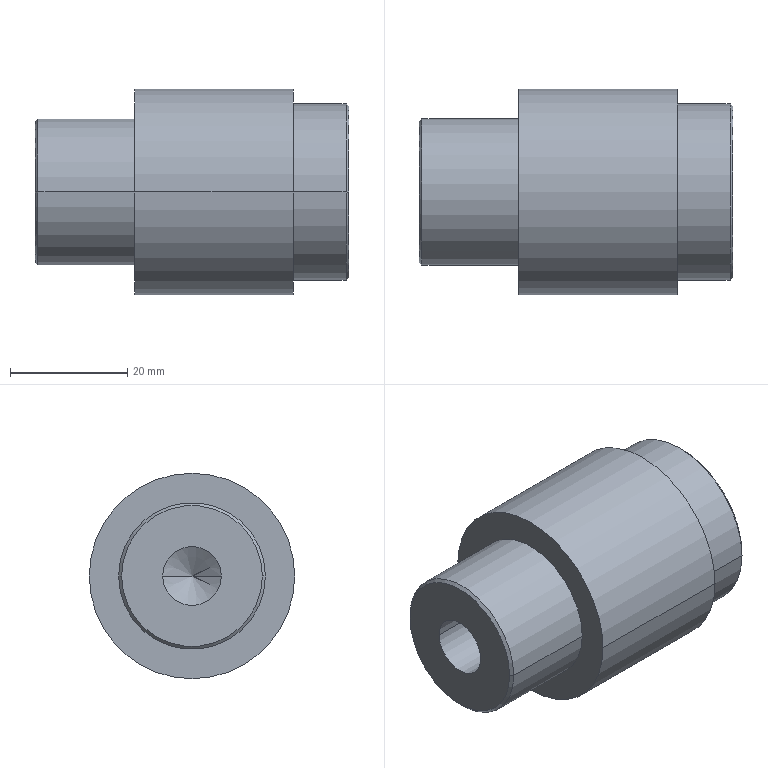Component | SolidWorks | GuideWheelAssembly-1_GuideWheelBracket-1_GuideWheelAxis-1 | 1 solid | 18 faces | box 53.5 x 35 x 35 mm | volume 39013 mm3 | cylinder 8 | cone 6 | plane 4 | commonest cylinder face diameters 10 x2 25 x2 35 x2 30 x2 | material Nylon 101
build123d program:
from build123d import *

# Parameters (mm, degrees)
SKETCH2_R              = 15
BOSS_EXTRUDE1_DEPTH    = 9.5
SKETCH3_R              = 17.5
BOSS_EXTRUDE2_DEPTH    = 27
SKETCH4_R              = 12.5
BOSS_EXTRUDE3_DEPTH    = 17
CHAMFER1_SIZE          = 0.5
M10_TAPPED_HOLE1_D     = 10
M10_TAPPED_HOLE1_DEPTH = 24.5
M10_TAPPED_HOLE1_TIP   = 3.004


with BuildPart() as part:
    # Sketch2 → Boss-Extrude1 (new body)
    with BuildSketch(Plane.XY):
        Circle(SKETCH2_R)
    extrude(amount=BOSS_EXTRUDE1_DEPTH)

    # Sketch3 → Boss-Extrude2 (add)
    with BuildSketch(Plane.XY.offset(9.5)):
        Circle(SKETCH3_R)
    extrude(amount=BOSS_EXTRUDE2_DEPTH)

    # Sketch4 → Boss-Extrude3 (add)
    with BuildSketch(Plane.XY.offset(36.5)):
        Circle(SKETCH4_R)
    extrude(amount=BOSS_EXTRUDE3_DEPTH)

    # Chamfer1
    chamfer1_edges = [part.edges().sort_by_distance(p)[0] for p in [
        (-12.5, 0, 53.5),
        (-15, 0, 0),
    ]]
    chamfer(chamfer1_edges, length=CHAMFER1_SIZE)

    # M10 Tapped Hole1
    with Locations(Plane.XY.offset(53.5)):
        with Locations((0, 0)):
            Hole(M10_TAPPED_HOLE1_D / 2, depth=M10_TAPPED_HOLE1_DEPTH)
            with Locations((0, 0, -(M10_TAPPED_HOLE1_DEPTH + M10_TAPPED_HOLE1_TIP / 2))):  # 118° drill point
                Cone(0, M10_TAPPED_HOLE1_D / 2, M10_TAPPED_HOLE1_TIP, mode=Mode.SUBTRACT)


solid = part.part

# Placed as in the assembly
solid = solid.moved(Location((-510.5, 0, 25), (0, -90, 0)))
STEP:
#1=COLOUR_RGB('',0.7922,0.8196,0.9333);
#2=FILL_AREA_STYLE_COLOUR('',#1);
#3=FILL_AREA_STYLE('',(#2));
#4=SURFACE_STYLE_FILL_AREA(#3);
#5=SURFACE_SIDE_STYLE('',(#4));
#6=SURFACE_STYLE_USAGE(.BOTH.,#5);
#7=PRESENTATION_STYLE_ASSIGNMENT((#6));
#8=CARTESIAN_POINT('',(-21.24,0.1969,0.9843));
#9=VERTEX_POINT('',#8);
#10=CARTESIAN_POINT('',(-21.24,-0.1969,0.9843));
#11=VERTEX_POINT('',#10);
#12=CARTESIAN_POINT('',(-21.24,-0.,0.9843));
#13=DIRECTION('',(-1.,0.,0.));
#14=DIRECTION('',(0.,-1.,0.));
#15=AXIS2_PLACEMENT_3D('',#12,#13,#14);
#16=CIRCLE('',#15,0.1969);
#17=EDGE_CURVE('',#9,#11,#16,.T.);
#18=ORIENTED_EDGE('',*,*,#17,.F.);
#19=CARTESIAN_POINT('',(-22.205,0.1969,0.9843));
#20=VERTEX_POINT('',#19);
#21=CARTESIAN_POINT('',(-22.205,0.1969,0.9843));
#22=DIRECTION('',(-1.,0.,0.));
#23=VECTOR('',#22,39.37);
#24=LINE('',#21,#23);
#25=EDGE_CURVE('',#9,#20,#24,.T.);
#26=ORIENTED_EDGE('',*,*,#25,.T.);
#27=CARTESIAN_POINT('',(-22.205,-0.1969,0.9843));
#28=VERTEX_POINT('',#27);
#29=CARTESIAN_POINT('',(-22.205,-0.,0.9843));
#30=DIRECTION('',(-1.,0.,0.));
#31=DIRECTION('',(0.,-1.,0.));
#32=AXIS2_PLACEMENT_3D('',#29,#30,#31);
#33=CIRCLE('',#32,0.1969);
#34=EDGE_CURVE('',#20,#28,#33,.T.);
#35=ORIENTED_EDGE('',*,*,#34,.T.);
#36=CARTESIAN_POINT('',(-22.205,-0.1969,0.9843));
#37=DIRECTION('',(-1.,0.,0.));
#38=VECTOR('',#37,39.37);
#39=LINE('',#36,#38);
#40=EDGE_CURVE('',#11,#28,#39,.T.);
#41=ORIENTED_EDGE('',*,*,#40,.F.);
#42=EDGE_LOOP('',(#18,#26,#35,#41));
#43=FACE_OUTER_BOUND('',#42,.T.);
#44=CARTESIAN_POINT('',(-22.205,-0.,0.9843));
#45=DIRECTION('',(-1.,0.,0.));
#46=DIRECTION('',(0.,-1.,0.));
#47=AXIS2_PLACEMENT_3D('',#44,#45,#46);
#48=CYLINDRICAL_SURFACE('',#47,0.1969);
#49=ADVANCED_FACE('',(#43),#48,.F.);
#50=CARTESIAN_POINT('',(-21.122,-0.,0.9843));
#51=VERTEX_POINT('',#50);
#52=CARTESIAN_POINT('',(-21.24,-0.1969,0.9843));
#53=DIRECTION('',(-0.515,-0.8572,0.));
#54=VECTOR('',#53,39.37);
#55=LINE('',#52,#54);
#56=EDGE_CURVE('',#51,#11,#55,.T.);
#57=ORIENTED_EDGE('',*,*,#56,.F.);
#58=CARTESIAN_POINT('',(-21.24,0.1969,0.9843));
#59=DIRECTION('',(-0.515,0.8572,0.));
#60=VECTOR('',#59,39.37);
#61=LINE('',#58,#60);
#62=EDGE_CURVE('',#51,#9,#61,.T.);
#63=ORIENTED_EDGE('',*,*,#62,.T.);
#64=ORIENTED_EDGE('',*,*,#17,.T.);
#65=EDGE_LOOP('',(#57,#63,#64));
#66=FACE_OUTER_BOUND('',#65,.T.);
#67=CARTESIAN_POINT('',(-21.24,-0.,0.9843));
#68=DIRECTION('',(-1.,0.,0.));
#69=DIRECTION('',(0.,-1.,0.));
#70=AXIS2_PLACEMENT_3D('',#67,#68,#69);
#71=CONICAL_SURFACE('',#70,0.1969,1.03);
#72=ADVANCED_FACE('',(#66),#71,.F.);
#73=CARTESIAN_POINT('',(-22.205,-0.4724,0.9843));
#74=VERTEX_POINT('',#73);
#75=CARTESIAN_POINT('',(-22.205,0.4724,0.9843));
#76=VERTEX_POINT('',#75);
#77=CARTESIAN_POINT('',(-22.205,-0.,0.9843));
#78=DIRECTION('',(-1.,0.,0.));
#79=DIRECTION('',(0.,-1.,0.));
#80=AXIS2_PLACEMENT_3D('',#77,#78,#79);
#81=CIRCLE('',#80,0.4724);
#82=EDGE_CURVE('',#74,#76,#81,.T.);
#83=ORIENTED_EDGE('',*,*,#82,.F.);
#84=CARTESIAN_POINT('',(-22.185,-0.4921,0.9843));
#85=VERTEX_POINT('',#84);
#86=CARTESIAN_POINT('',(-22.205,-0.4724,0.9843));
#87=DIRECTION('',(0.7071,-0.7071,0.));
#88=VECTOR('',#87,39.37);
#89=LINE('',#86,#88);
#90=EDGE_CURVE('',#74,#85,#89,.T.);
#91=ORIENTED_EDGE('',*,*,#90,.T.);
#92=CARTESIAN_POINT('',(-22.185,0.4921,0.9843));
#93=VERTEX_POINT('',#92);
#94=CARTESIAN_POINT('',(-22.185,-0.,0.9843));
#95=DIRECTION('',(1.,0.,0.));
#96=DIRECTION('',(0.,-1.,0.));
#97=AXIS2_PLACEMENT_3D('',#94,#95,#96);
#98=CIRCLE('',#97,0.4921);
#99=EDGE_CURVE('',#93,#85,#98,.T.);
#100=ORIENTED_EDGE('',*,*,#99,.F.);
#101=CARTESIAN_POINT('',(-22.205,0.4724,0.9843));
#102=DIRECTION('',(0.7071,0.7071,-0.));
#103=VECTOR('',#102,39.37);
#104=LINE('',#101,#103);
#105=EDGE_CURVE('',#76,#93,#104,.T.);
#106=ORIENTED_EDGE('',*,*,#105,.F.);
#107=EDGE_LOOP('',(#83,#91,#100,#106));
#108=FACE_OUTER_BOUND('',#107,.T.);
#109=CARTESIAN_POINT('',(-22.205,-0.,0.9843));
#110=DIRECTION('',(1.,0.,0.));
#111=DIRECTION('',(0.,1.,0.));
#112=AXIS2_PLACEMENT_3D('',#109,#110,#111);
#113=CONICAL_SURFACE('',#112,0.4724,0.7854);
#114=ADVANCED_FACE('',(#108),#113,.T.);
#115=CARTESIAN_POINT('',(-20.098,0.5709,0.9843));
#116=VERTEX_POINT('',#115);
#117=CARTESIAN_POINT('',(-20.098,-0.5709,0.9843));
#118=VERTEX_POINT('',#117);
#119=CARTESIAN_POINT('',(-20.098,-0.,0.9843));
#120=DIRECTION('',(1.,0.,0.));
#121=DIRECTION('',(0.,-1.,0.));
#122=AXIS2_PLACEMENT_3D('',#119,#120,#121);
#123=CIRCLE('',#122,0.5709);
#124=EDGE_CURVE('',#116,#118,#123,.T.);
#125=ORIENTED_EDGE('',*,*,#124,.F.);
#126=CARTESIAN_POINT('',(-20.118,0.5906,0.9843));
#127=VERTEX_POINT('',#126);
#128=CARTESIAN_POINT('',(-20.118,0.5906,0.9843));
#129=DIRECTION('',(-0.7071,0.7071,0.));
#130=VECTOR('',#129,39.37);
#131=LINE('',#128,#130);
#132=EDGE_CURVE('',#116,#127,#131,.T.);
#133=ORIENTED_EDGE('',*,*,#132,.T.);
#134=CARTESIAN_POINT('',(-20.118,-0.5906,0.9843));
#135=VERTEX_POINT('',#134);
#136=CARTESIAN_POINT('',(-20.118,-0.,0.9843));
#137=DIRECTION('',(-1.,0.,0.));
#138=DIRECTION('',(0.,-1.,0.));
#139=AXIS2_PLACEMENT_3D('',#136,#137,#138);
#140=CIRCLE('',#139,0.5906);
#141=EDGE_CURVE('',#135,#127,#140,.T.);
#142=ORIENTED_EDGE('',*,*,#141,.F.);
#143=CARTESIAN_POINT('',(-20.118,-0.5906,0.9843));
#144=DIRECTION('',(-0.7071,-0.7071,0.));
#145=VECTOR('',#144,39.37);
#146=LINE('',#143,#145);
#147=EDGE_CURVE('',#118,#135,#146,.T.);
#148=ORIENTED_EDGE('',*,*,#147,.F.);
#149=EDGE_LOOP('',(#125,#133,#142,#148));
#150=FACE_OUTER_BOUND('',#149,.T.);
#151=CARTESIAN_POINT('',(-20.118,-0.,0.9843));
#152=DIRECTION('',(-1.,0.,0.));
#153=DIRECTION('',(0.,-1.,0.));
#154=AXIS2_PLACEMENT_3D('',#151,#152,#153);
#155=CONICAL_SURFACE('',#154,0.5906,0.7854);
#156=ADVANCED_FACE('',(#150),#155,.T.);
#157=ORIENTED_EDGE('',*,*,#99,.T.);
#158=CARTESIAN_POINT('',(-21.535,-0.4921,0.9843));
#159=VERTEX_POINT('',#158);
#160=CARTESIAN_POINT('',(-22.205,-0.4921,0.9843));
#161=DIRECTION('',(1.,0.,0.));
#162=VECTOR('',#161,39.37);
#163=LINE('',#160,#162);
#164=EDGE_CURVE('',#85,#159,#163,.T.);
#165=ORIENTED_EDGE('',*,*,#164,.T.);
#166=CARTESIAN_POINT('',(-21.535,0.4921,0.9843));
#167=VERTEX_POINT('',#166);
#168=CARTESIAN_POINT('',(-21.535,-0.,0.9843));
#169=DIRECTION('',(-1.,0.,0.));
#170=DIRECTION('',(0.,-1.,0.));
#171=AXIS2_PLACEMENT_3D('',#168,#169,#170);
#172=CIRCLE('',#171,0.4921);
#173=EDGE_CURVE('',#159,#167,#172,.T.);
#174=ORIENTED_EDGE('',*,*,#173,.T.);
#175=CARTESIAN_POINT('',(-22.205,0.4921,0.9843));
#176=DIRECTION('',(1.,0.,0.));
#177=VECTOR('',#176,39.37);
#178=LINE('',#175,#177);
#179=EDGE_CURVE('',#93,#167,#178,.T.);
#180=ORIENTED_EDGE('',*,*,#179,.F.);
#181=EDGE_LOOP('',(#157,#165,#174,#180));
#182=FACE_OUTER_BOUND('',#181,.T.);
#183=CARTESIAN_POINT('',(-22.205,-0.,0.9843));
#184=DIRECTION('',(1.,0.,0.));
#185=DIRECTION('',(0.,1.,0.));
#186=AXIS2_PLACEMENT_3D('',#183,#184,#185);
#187=CYLINDRICAL_SURFACE('',#186,0.4921);
#188=ADVANCED_FACE('',(#182),#187,.T.);
#189=CARTESIAN_POINT('',(-21.535,-0.689,0.9843));
#190=VERTEX_POINT('',#189);
#191=CARTESIAN_POINT('',(-21.535,0.689,0.9843));
#192=VERTEX_POINT('',#191);
#193=CARTESIAN_POINT('',(-21.535,-0.,0.9843));
#194=DIRECTION('',(-1.,0.,0.));
#195=DIRECTION('',(0.,-1.,0.));
#196=AXIS2_PLACEMENT_3D('',#193,#194,#195);
#197=CIRCLE('',#196,0.689);
#198=EDGE_CURVE('',#190,#192,#197,.T.);
#199=ORIENTED_EDGE('',*,*,#198,.F.);
#200=CARTESIAN_POINT('',(-20.472,-0.689,0.9843));
#201=VERTEX_POINT('',#200);
#202=CARTESIAN_POINT('',(-21.535,-0.689,0.9843));
#203=DIRECTION('',(1.,0.,0.));
#204=VECTOR('',#203,39.37);
#205=LINE('',#202,#204);
#206=EDGE_CURVE('',#190,#201,#205,.T.);
#207=ORIENTED_EDGE('',*,*,#206,.T.);
#208=CARTESIAN_POINT('',(-20.472,0.689,0.9843));
#209=VERTEX_POINT('',#208);
#210=CARTESIAN_POINT('',(-20.472,-0.,0.9843));
#211=DIRECTION('',(-1.,0.,0.));
#212=DIRECTION('',(0.,-1.,0.));
#213=AXIS2_PLACEMENT_3D('',#210,#211,#212);
#214=CIRCLE('',#213,0.689);
#215=EDGE_CURVE('',#201,#209,#214,.T.);
#216=ORIENTED_EDGE('',*,*,#215,.T.);
#217=CARTESIAN_POINT('',(-21.535,0.689,0.9843));
#218=DIRECTION('',(1.,0.,0.));
#219=VECTOR('',#218,39.37);
#220=LINE('',#217,#219);
#221=EDGE_CURVE('',#192,#209,#220,.T.);
#222=ORIENTED_EDGE('',*,*,#221,.F.);
#223=EDGE_LOOP('',(#199,#207,#216,#222));
#224=FACE_OUTER_BOUND('',#223,.T.);
#225=CARTESIAN_POINT('',(-21.535,-0.,0.9843));
#226=DIRECTION('',(1.,0.,0.));
#227=DIRECTION('',(0.,1.,-0.));
#228=AXIS2_PLACEMENT_3D('',#225,#226,#227);
#229=CYLINDRICAL_SURFACE('',#228,0.689);
#230=ADVANCED_FACE('',(#224),#229,.T.);
#231=CARTESIAN_POINT('',(-20.472,-0.5906,0.9843));
#232=VERTEX_POINT('',#231);
#233=CARTESIAN_POINT('',(-20.472,0.5906,0.9843));
#234=VERTEX_POINT('',#233);
#235=CARTESIAN_POINT('',(-20.472,-0.,0.9843));
#236=DIRECTION('',(-1.,0.,0.));
#237=DIRECTION('',(0.,-1.,0.));
#238=AXIS2_PLACEMENT_3D('',#235,#236,#237);
#239=CIRCLE('',#238,0.5906);
#240=EDGE_CURVE('',#232,#234,#239,.T.);
#241=ORIENTED_EDGE('',*,*,#240,.F.);
#242=CARTESIAN_POINT('',(-20.472,-0.5906,0.9843));
#243=DIRECTION('',(1.,0.,0.));
#244=VECTOR('',#243,39.37);
#245=LINE('',#242,#244);
#246=EDGE_CURVE('',#232,#135,#245,.T.);
#247=ORIENTED_EDGE('',*,*,#246,.T.);
#248=ORIENTED_EDGE('',*,*,#141,.T.);
#249=CARTESIAN_POINT('',(-20.472,0.5906,0.9843));
#250=DIRECTION('',(1.,0.,0.));
#251=VECTOR('',#250,39.37);
#252=LINE('',#249,#251);
#253=EDGE_CURVE('',#234,#127,#252,.T.);
#254=ORIENTED_EDGE('',*,*,#253,.F.);
#255=EDGE_LOOP('',(#241,#247,#248,#254));
#256=FACE_OUTER_BOUND('',#255,.T.);
#257=CARTESIAN_POINT('',(-20.472,-0.,0.9843));
#258=DIRECTION('',(1.,0.,0.));
#259=DIRECTION('',(0.,1.,0.));
#260=AXIS2_PLACEMENT_3D('',#257,#258,#259);
#261=CYLINDRICAL_SURFACE('',#260,0.5906);
#262=ADVANCED_FACE('',(#256),#261,.T.);
#263=CARTESIAN_POINT('',(-21.535,-0.,0.9843));
#264=DIRECTION('',(-1.,0.,0.));
#265=DIRECTION('',(0.,-1.,0.));
#266=AXIS2_PLACEMENT_3D('',#263,#264,#265);
#267=CIRCLE('',#266,0.689);
#268=EDGE_CURVE('',#192,#190,#267,.T.);
#269=ORIENTED_EDGE('',*,*,#268,.T.);
#270=ORIENTED_EDGE('',*,*,#198,.T.);
#271=EDGE_LOOP('',(#269,#270));
#272=FACE_OUTER_BOUND('',#271,.T.);
#273=CARTESIAN_POINT('',(-21.535,-0.,0.9843));
#274=DIRECTION('',(-1.,0.,0.));
#275=DIRECTION('',(0.,-1.,0.));
#276=AXIS2_PLACEMENT_3D('',#273,#274,#275);
#277=CIRCLE('',#276,0.4921);
#278=EDGE_CURVE('',#167,#159,#277,.T.);
#279=ORIENTED_EDGE('',*,*,#278,.F.);
#280=ORIENTED_EDGE('',*,*,#173,.F.);
#281=EDGE_LOOP('',(#279,#280));
#282=FACE_BOUND('',#281,.T.);
#283=CARTESIAN_POINT('',(-21.535,-0.,0.9843));
#284=DIRECTION('',(-1.,0.,0.));
#285=DIRECTION('',(0.,-1.,0.));
#286=AXIS2_PLACEMENT_3D('',#283,#284,#285);
#287=PLANE('',#286);
#288=ADVANCED_FACE('',(#272,#282),#287,.T.);
#289=ORIENTED_EDGE('',*,*,#246,.F.);
#290=CARTESIAN_POINT('',(-20.472,-0.,0.9843));
#291=DIRECTION('',(-1.,0.,0.));
#292=DIRECTION('',(0.,-1.,0.));
#293=AXIS2_PLACEMENT_3D('',#290,#291,#292);
#294=CIRCLE('',#293,0.5906);
#295=EDGE_CURVE('',#234,#232,#294,.T.);
#296=ORIENTED_EDGE('',*,*,#295,.F.);
#297=ORIENTED_EDGE('',*,*,#253,.T.);
#298=CARTESIAN_POINT('',(-20.118,-0.,0.9843));
#299=DIRECTION('',(-1.,0.,0.));
#300=DIRECTION('',(0.,-1.,0.));
#301=AXIS2_PLACEMENT_3D('',#298,#299,#300);
#302=CIRCLE('',#301,0.5906);
#303=EDGE_CURVE('',#127,#135,#302,.T.);
#304=ORIENTED_EDGE('',*,*,#303,.T.);
#305=EDGE_LOOP('',(#289,#296,#297,#304));
#306=FACE_OUTER_BOUND('',#305,.T.);
#307=CARTESIAN_POINT('',(-20.472,-0.,0.9843));
#308=DIRECTION('',(1.,0.,0.));
#309=DIRECTION('',(0.,1.,0.));
#310=AXIS2_PLACEMENT_3D('',#307,#308,#309);
#311=CYLINDRICAL_SURFACE('',#310,0.5906);
#312=ADVANCED_FACE('',(#306),#311,.T.);
#313=CARTESIAN_POINT('',(-20.098,-0.,0.9843));
#314=DIRECTION('',(1.,0.,0.));
#315=DIRECTION('',(0.,-1.,0.));
#316=AXIS2_PLACEMENT_3D('',#313,#314,#315);
#317=CIRCLE('',#316,0.5709);
#318=EDGE_CURVE('',#118,#116,#317,.T.);
#319=ORIENTED_EDGE('',*,*,#318,.T.);
#320=ORIENTED_EDGE('',*,*,#124,.T.);
#321=EDGE_LOOP('',(#319,#320));
#322=FACE_OUTER_BOUND('',#321,.T.);
#323=CARTESIAN_POINT('',(-20.098,-0.,0.9843));
#324=DIRECTION('',(-1.,0.,0.));
#325=DIRECTION('',(0.,-1.,0.));
#326=AXIS2_PLACEMENT_3D('',#323,#324,#325);
#327=PLANE('',#326);
#328=ADVANCED_FACE('',(#322),#327,.F.);
#329=CARTESIAN_POINT('',(-20.472,-0.,0.9843));
#330=DIRECTION('',(-1.,0.,0.));
#331=DIRECTION('',(0.,-1.,0.));
#332=AXIS2_PLACEMENT_3D('',#329,#330,#331);
#333=CIRCLE('',#332,0.689);
#334=EDGE_CURVE('',#209,#201,#333,.T.);
#335=ORIENTED_EDGE('',*,*,#334,.F.);
#336=ORIENTED_EDGE('',*,*,#215,.F.);
#337=EDGE_LOOP('',(#335,#336));
#338=FACE_OUTER_BOUND('',#337,.T.);
#339=ORIENTED_EDGE('',*,*,#295,.T.);
#340=ORIENTED_EDGE('',*,*,#240,.T.);
#341=EDGE_LOOP('',(#339,#340));
#342=FACE_BOUND('',#341,.T.);
#343=CARTESIAN_POINT('',(-20.472,-0.,0.9843));
#344=DIRECTION('',(-1.,0.,0.));
#345=DIRECTION('',(0.,-1.,0.));
#346=AXIS2_PLACEMENT_3D('',#343,#344,#345);
#347=PLANE('',#346);
#348=ADVANCED_FACE('',(#338,#342),#347,.F.);
#349=ORIENTED_EDGE('',*,*,#206,.F.);
#350=ORIENTED_EDGE('',*,*,#268,.F.);
#351=ORIENTED_EDGE('',*,*,#221,.T.);
#352=ORIENTED_EDGE('',*,*,#334,.T.);
#353=EDGE_LOOP('',(#349,#350,#351,#352));
#354=FACE_OUTER_BOUND('',#353,.T.);
#355=CARTESIAN_POINT('',(-21.535,-0.,0.9843));
#356=DIRECTION('',(1.,0.,0.));
#357=DIRECTION('',(0.,1.,-0.));
#358=AXIS2_PLACEMENT_3D('',#355,#356,#357);
#359=CYLINDRICAL_SURFACE('',#358,0.689);
#360=ADVANCED_FACE('',(#354),#359,.T.);
#361=ORIENTED_EDGE('',*,*,#164,.F.);
#362=CARTESIAN_POINT('',(-22.185,-0.,0.9843));
#363=DIRECTION('',(1.,0.,0.));
#364=DIRECTION('',(0.,-1.,0.));
#365=AXIS2_PLACEMENT_3D('',#362,#363,#364);
#366=CIRCLE('',#365,0.4921);
#367=EDGE_CURVE('',#85,#93,#366,.T.);
#368=ORIENTED_EDGE('',*,*,#367,.T.);
#369=ORIENTED_EDGE('',*,*,#179,.T.);
#370=ORIENTED_EDGE('',*,*,#278,.T.);
#371=EDGE_LOOP('',(#361,#368,#369,#370));
#372=FACE_OUTER_BOUND('',#371,.T.);
#373=CARTESIAN_POINT('',(-22.205,-0.,0.9843));
#374=DIRECTION('',(1.,0.,0.));
#375=DIRECTION('',(0.,1.,0.));
#376=AXIS2_PLACEMENT_3D('',#373,#374,#375);
#377=CYLINDRICAL_SURFACE('',#376,0.4921);
#378=ADVANCED_FACE('',(#372),#377,.T.);
#379=CARTESIAN_POINT('',(-22.205,-0.,0.9843));
#380=DIRECTION('',(-1.,0.,0.));
#381=DIRECTION('',(0.,-1.,0.));
#382=AXIS2_PLACEMENT_3D('',#379,#380,#381);
#383=CIRCLE('',#382,0.1969);
#384=EDGE_CURVE('',#28,#20,#383,.T.);
#385=ORIENTED_EDGE('',*,*,#384,.F.);
#386=ORIENTED_EDGE('',*,*,#34,.F.);
#387=EDGE_LOOP('',(#385,#386));
#388=FACE_BOUND('',#387,.T.);
#389=CARTESIAN_POINT('',(-22.205,-0.,0.9843));
#390=DIRECTION('',(-1.,0.,0.));
#391=DIRECTION('',(0.,-1.,0.));
#392=AXIS2_PLACEMENT_3D('',#389,#390,#391);
#393=CIRCLE('',#392,0.4724);
#394=EDGE_CURVE('',#76,#74,#393,.T.);
#395=ORIENTED_EDGE('',*,*,#394,.T.);
#396=ORIENTED_EDGE('',*,*,#82,.T.);
#397=EDGE_LOOP('',(#395,#396));
#398=FACE_OUTER_BOUND('',#397,.T.);
#399=CARTESIAN_POINT('',(-22.205,-0.,0.9843));
#400=DIRECTION('',(-1.,0.,0.));
#401=DIRECTION('',(0.,-1.,0.));
#402=AXIS2_PLACEMENT_3D('',#399,#400,#401);
#403=PLANE('',#402);
#404=ADVANCED_FACE('',(#388,#398),#403,.T.);
#405=ORIENTED_EDGE('',*,*,#132,.F.);
#406=ORIENTED_EDGE('',*,*,#318,.F.);
#407=ORIENTED_EDGE('',*,*,#147,.T.);
#408=ORIENTED_EDGE('',*,*,#303,.F.);
#409=EDGE_LOOP('',(#405,#406,#407,#408));
#410=FACE_OUTER_BOUND('',#409,.T.);
#411=CARTESIAN_POINT('',(-20.118,-0.,0.9843));
#412=DIRECTION('',(-1.,0.,0.));
#413=DIRECTION('',(0.,-1.,0.));
#414=AXIS2_PLACEMENT_3D('',#411,#412,#413);
#415=CONICAL_SURFACE('',#414,0.5906,0.7854);
#416=ADVANCED_FACE('',(#410),#415,.T.);
#417=ORIENTED_EDGE('',*,*,#90,.F.);
#418=ORIENTED_EDGE('',*,*,#394,.F.);
#419=ORIENTED_EDGE('',*,*,#105,.T.);
#420=ORIENTED_EDGE('',*,*,#367,.F.);
#421=EDGE_LOOP('',(#417,#418,#419,#420));
#422=FACE_OUTER_BOUND('',#421,.T.);
#423=CARTESIAN_POINT('',(-22.205,-0.,0.9843));
#424=DIRECTION('',(1.,0.,0.));
#425=DIRECTION('',(0.,1.,0.));
#426=AXIS2_PLACEMENT_3D('',#423,#424,#425);
#427=CONICAL_SURFACE('',#426,0.4724,0.7854);
#428=ADVANCED_FACE('',(#422),#427,.T.);
#429=ORIENTED_EDGE('',*,*,#62,.F.);
#430=ORIENTED_EDGE('',*,*,#56,.T.);
#431=CARTESIAN_POINT('',(-21.24,-0.,0.9843));
#432=DIRECTION('',(-1.,0.,0.));
#433=DIRECTION('',(0.,-1.,0.));
#434=AXIS2_PLACEMENT_3D('',#431,#432,#433);
#435=CIRCLE('',#434,0.1969);
#436=EDGE_CURVE('',#11,#9,#435,.T.);
#437=ORIENTED_EDGE('',*,*,#436,.T.);
#438=EDGE_LOOP('',(#429,#430,#437));
#439=FACE_OUTER_BOUND('',#438,.T.);
#440=CARTESIAN_POINT('',(-21.24,-0.,0.9843));
#441=DIRECTION('',(-1.,0.,0.));
#442=DIRECTION('',(0.,-1.,0.));
#443=AXIS2_PLACEMENT_3D('',#440,#441,#442);
#444=CONICAL_SURFACE('',#443,0.1969,1.03);
#445=ADVANCED_FACE('',(#439),#444,.F.);
#446=ORIENTED_EDGE('',*,*,#25,.F.);
#447=ORIENTED_EDGE('',*,*,#436,.F.);
#448=ORIENTED_EDGE('',*,*,#40,.T.);
#449=ORIENTED_EDGE('',*,*,#384,.T.);
#450=EDGE_LOOP('',(#446,#447,#448,#449));
#451=FACE_OUTER_BOUND('',#450,.T.);
#452=CARTESIAN_POINT('',(-22.205,-0.,0.9843));
#453=DIRECTION('',(-1.,0.,0.));
#454=DIRECTION('',(0.,-1.,0.));
#455=AXIS2_PLACEMENT_3D('',#452,#453,#454);
#456=CYLINDRICAL_SURFACE('',#455,0.1969);
#457=ADVANCED_FACE('',(#451),#456,.F.);
#458=CLOSED_SHELL('',(#49,#72,#114,#156,#188,#230,#262,#288,#312,#328,#348,#360,#378,#404,#416,#428,#445,#457));
#459=MANIFOLD_SOLID_BREP('',#458);
#460=STYLED_ITEM('',(#7),#459);
#461=(LENGTH_UNIT()NAMED_UNIT(*)SI_UNIT($,.METRE.));
#462=LENGTH_MEASURE_WITH_UNIT(LENGTH_MEASURE(0.0254),#461);
#463=DIMENSIONAL_EXPONENTS(1.,0.,0.,0.,0.,0.,0.);
#464=(CONVERSION_BASED_UNIT('',#462)LENGTH_UNIT()NAMED_UNIT(#463));
#465=UNCERTAINTY_MEASURE_WITH_UNIT(LENGTH_MEASURE(0.00001),#464,'','');
#466=(NAMED_UNIT(*)PLANE_ANGLE_UNIT()SI_UNIT($,.RADIAN.));
#467=(NAMED_UNIT(*)SI_UNIT($,.STERADIAN.)SOLID_ANGLE_UNIT());
#468=(GEOMETRIC_REPRESENTATION_CONTEXT(3)GLOBAL_UNCERTAINTY_ASSIGNED_CONTEXT((#465))GLOBAL_UNIT_ASSIGNED_CONTEXT((#464,#466,#467))REPRESENTATION_CONTEXT('',''));
#469=MECHANICAL_DESIGN_GEOMETRIC_PRESENTATION_REPRESENTATION('',(#460),#468);
#470=PRESENTATION_LAYER_ASSIGNMENT('','',(#460));
#471=CARTESIAN_POINT('',(0.,0.,0.));
#472=DIRECTION('',(0.,0.,1.));
#473=DIRECTION('',(1.,0.,0.));
#474=AXIS2_PLACEMENT_3D('',#471,#472,#473);
#475=(LENGTH_UNIT()NAMED_UNIT(*)SI_UNIT($,.METRE.));
#476=LENGTH_MEASURE_WITH_UNIT(LENGTH_MEASURE(0.0254),#475);
#477=DIMENSIONAL_EXPONENTS(1.,0.,0.,0.,0.,0.,0.);
#478=(CONVERSION_BASED_UNIT('',#476)LENGTH_UNIT()NAMED_UNIT(#477));
#479=UNCERTAINTY_MEASURE_WITH_UNIT(LENGTH_MEASURE(0.00001),#478,'','');
#480=(NAMED_UNIT(*)PLANE_ANGLE_UNIT()SI_UNIT($,.RADIAN.));
#481=(NAMED_UNIT(*)SI_UNIT($,.STERADIAN.)SOLID_ANGLE_UNIT());
#482=(GEOMETRIC_REPRESENTATION_CONTEXT(3)GLOBAL_UNCERTAINTY_ASSIGNED_CONTEXT((#479))GLOBAL_UNIT_ASSIGNED_CONTEXT((#478,#480,#481))REPRESENTATION_CONTEXT('',''));
#483=ADVANCED_BREP_SHAPE_REPRESENTATION('',(#459,#474),#482);